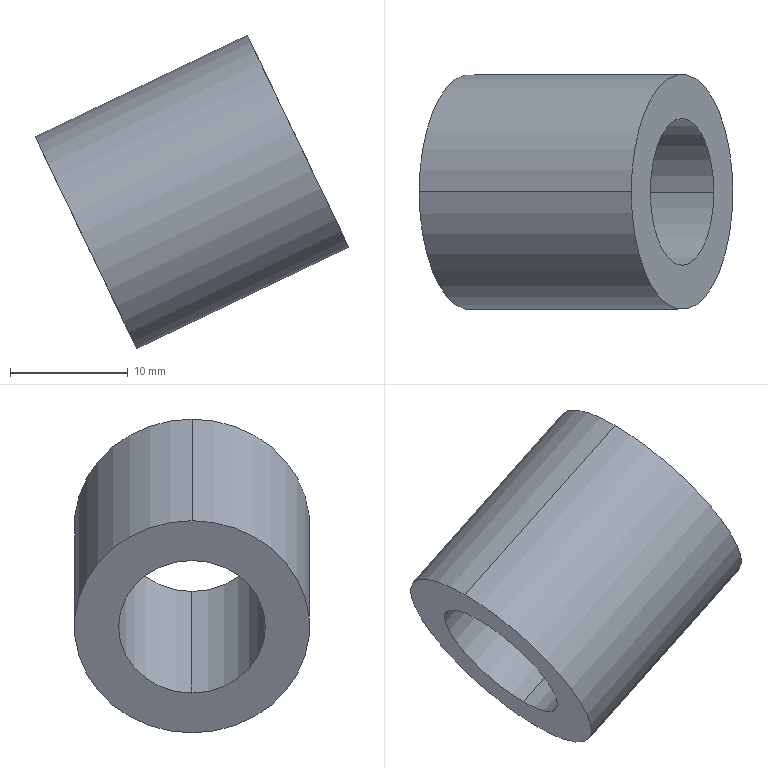Component | SolidWorks | Washer1-1-2 | 1 solid | 6 faces | box 26.68 x 20 x 26.68 mm | volume 3829 mm3 | cylinder 4 | plane 2 | commonest cylinder face diameters 12.5 x2 20 x2
build123d program:
from build123d import *

# Parameters (mm, degrees)
SKETCH1_R           = 10
SKETCH1_R_2         = 6.25
BOSS_EXTRUDE1_DEPTH = 20


with BuildPart() as part:
    # Sketch1 → Boss-Extrude1 (new body)
    with BuildSketch(Plane.XY):
        Circle(SKETCH1_R)
        Circle(SKETCH1_R_2, mode=Mode.SUBTRACT)
    extrude(amount=BOSS_EXTRUDE1_DEPTH)


solid = part.part

# Placed as in the assembly
solid = solid.moved(Location((-95.293, 250, 667.757), (0, 64.419, 168.667)))
STEP:
#1=COLOUR_RGB('',0.7922,0.8196,0.9333);
#2=FILL_AREA_STYLE_COLOUR('',#1);
#3=FILL_AREA_STYLE('',(#2));
#4=SURFACE_STYLE_FILL_AREA(#3);
#5=SURFACE_SIDE_STYLE('',(#4));
#6=SURFACE_STYLE_USAGE(.BOTH.,#5);
#7=PRESENTATION_STYLE_ASSIGNMENT((#6));
#8=CARTESIAN_POINT('',(-3.148,9.843,26.852));
#9=VERTEX_POINT('',#8);
#10=CARTESIAN_POINT('',(-2.935,9.843,26.408));
#11=VERTEX_POINT('',#10);
#12=CARTESIAN_POINT('',(-3.041,9.843,26.63));
#13=DIRECTION('',(0.902,-0.,0.4318));
#14=DIRECTION('',(0.4318,0.,-0.902));
#15=AXIS2_PLACEMENT_3D('',#12,#13,#14);
#16=CIRCLE('',#15,0.2461);
#17=EDGE_CURVE('',#9,#11,#16,.T.);
#18=ORIENTED_EDGE('',*,*,#17,.T.);
#19=CARTESIAN_POINT('',(-3.645,9.843,26.068));
#20=VERTEX_POINT('',#19);
#21=CARTESIAN_POINT('',(-2.935,9.843,26.408));
#22=DIRECTION('',(-0.902,0.,-0.4318));
#23=VECTOR('',#22,39.37);
#24=LINE('',#21,#23);
#25=EDGE_CURVE('',#11,#20,#24,.T.);
#26=ORIENTED_EDGE('',*,*,#25,.T.);
#27=CARTESIAN_POINT('',(-3.858,9.843,26.512));
#28=VERTEX_POINT('',#27);
#29=CARTESIAN_POINT('',(-3.752,9.843,26.29));
#30=DIRECTION('',(0.902,-0.,0.4318));
#31=DIRECTION('',(0.4318,0.,-0.902));
#32=AXIS2_PLACEMENT_3D('',#29,#30,#31);
#33=CIRCLE('',#32,0.2461);
#34=EDGE_CURVE('',#28,#20,#33,.T.);
#35=ORIENTED_EDGE('',*,*,#34,.F.);
#36=CARTESIAN_POINT('',(-3.148,9.843,26.852));
#37=DIRECTION('',(-0.902,0.,-0.4318));
#38=VECTOR('',#37,39.37);
#39=LINE('',#36,#38);
#40=EDGE_CURVE('',#9,#28,#39,.T.);
#41=ORIENTED_EDGE('',*,*,#40,.F.);
#42=EDGE_LOOP('',(#18,#26,#35,#41));
#43=FACE_OUTER_BOUND('',#42,.T.);
#44=CARTESIAN_POINT('',(-3.041,9.843,26.63));
#45=DIRECTION('',(-0.902,0.,-0.4318));
#46=DIRECTION('',(-0.4318,-0.,0.902));
#47=AXIS2_PLACEMENT_3D('',#44,#45,#46);
#48=CYLINDRICAL_SURFACE('',#47,0.2461);
#49=ADVANCED_FACE('',(#43),#48,.F.);
#50=CARTESIAN_POINT('',(-2.871,9.843,26.275));
#51=VERTEX_POINT('',#50);
#52=CARTESIAN_POINT('',(-3.211,9.843,26.985));
#53=VERTEX_POINT('',#52);
#54=CARTESIAN_POINT('',(-3.041,9.843,26.63));
#55=DIRECTION('',(0.902,-0.,0.4318));
#56=DIRECTION('',(0.4318,0.,-0.902));
#57=AXIS2_PLACEMENT_3D('',#54,#55,#56);
#58=CIRCLE('',#57,0.3937);
#59=EDGE_CURVE('',#51,#53,#58,.T.);
#60=ORIENTED_EDGE('',*,*,#59,.F.);
#61=CARTESIAN_POINT('',(-3.582,9.843,25.935));
#62=VERTEX_POINT('',#61);
#63=CARTESIAN_POINT('',(-2.871,9.843,26.275));
#64=DIRECTION('',(-0.902,0.,-0.4318));
#65=VECTOR('',#64,39.37);
#66=LINE('',#63,#65);
#67=EDGE_CURVE('',#51,#62,#66,.T.);
#68=ORIENTED_EDGE('',*,*,#67,.T.);
#69=CARTESIAN_POINT('',(-3.922,9.843,26.645));
#70=VERTEX_POINT('',#69);
#71=CARTESIAN_POINT('',(-3.752,9.843,26.29));
#72=DIRECTION('',(0.902,-0.,0.4318));
#73=DIRECTION('',(0.4318,0.,-0.902));
#74=AXIS2_PLACEMENT_3D('',#71,#72,#73);
#75=CIRCLE('',#74,0.3937);
#76=EDGE_CURVE('',#62,#70,#75,.T.);
#77=ORIENTED_EDGE('',*,*,#76,.T.);
#78=CARTESIAN_POINT('',(-3.211,9.843,26.985));
#79=DIRECTION('',(-0.902,0.,-0.4318));
#80=VECTOR('',#79,39.37);
#81=LINE('',#78,#80);
#82=EDGE_CURVE('',#53,#70,#81,.T.);
#83=ORIENTED_EDGE('',*,*,#82,.F.);
#84=EDGE_LOOP('',(#60,#68,#77,#83));
#85=FACE_OUTER_BOUND('',#84,.T.);
#86=CARTESIAN_POINT('',(-3.041,9.843,26.63));
#87=DIRECTION('',(-0.902,0.,-0.4318));
#88=DIRECTION('',(-0.4318,-0.,0.902));
#89=AXIS2_PLACEMENT_3D('',#86,#87,#88);
#90=CYLINDRICAL_SURFACE('',#89,0.3937);
#91=ADVANCED_FACE('',(#85),#90,.T.);
#92=CARTESIAN_POINT('',(-3.041,9.843,26.63));
#93=DIRECTION('',(0.902,-0.,0.4318));
#94=DIRECTION('',(0.4318,0.,-0.902));
#95=AXIS2_PLACEMENT_3D('',#92,#93,#94);
#96=CIRCLE('',#95,0.3937);
#97=EDGE_CURVE('',#53,#51,#96,.T.);
#98=ORIENTED_EDGE('',*,*,#97,.T.);
#99=ORIENTED_EDGE('',*,*,#59,.T.);
#100=EDGE_LOOP('',(#98,#99));
#101=FACE_OUTER_BOUND('',#100,.T.);
#102=ORIENTED_EDGE('',*,*,#17,.F.);
#103=CARTESIAN_POINT('',(-3.041,9.843,26.63));
#104=DIRECTION('',(0.902,-0.,0.4318));
#105=DIRECTION('',(0.4318,0.,-0.902));
#106=AXIS2_PLACEMENT_3D('',#103,#104,#105);
#107=CIRCLE('',#106,0.2461);
#108=EDGE_CURVE('',#11,#9,#107,.T.);
#109=ORIENTED_EDGE('',*,*,#108,.F.);
#110=EDGE_LOOP('',(#102,#109));
#111=FACE_BOUND('',#110,.T.);
#112=CARTESIAN_POINT('',(-3.041,9.843,26.63));
#113=DIRECTION('',(0.902,-0.,0.4318));
#114=DIRECTION('',(0.4318,0.,-0.902));
#115=AXIS2_PLACEMENT_3D('',#112,#113,#114);
#116=PLANE('',#115);
#117=ADVANCED_FACE('',(#101,#111),#116,.T.);
#118=CARTESIAN_POINT('',(-3.752,9.843,26.29));
#119=DIRECTION('',(0.902,-0.,0.4318));
#120=DIRECTION('',(0.4318,0.,-0.902));
#121=AXIS2_PLACEMENT_3D('',#118,#119,#120);
#122=CIRCLE('',#121,0.3937);
#123=EDGE_CURVE('',#70,#62,#122,.T.);
#124=ORIENTED_EDGE('',*,*,#123,.F.);
#125=ORIENTED_EDGE('',*,*,#76,.F.);
#126=EDGE_LOOP('',(#124,#125));
#127=FACE_OUTER_BOUND('',#126,.T.);
#128=ORIENTED_EDGE('',*,*,#34,.T.);
#129=CARTESIAN_POINT('',(-3.752,9.843,26.29));
#130=DIRECTION('',(0.902,-0.,0.4318));
#131=DIRECTION('',(0.4318,0.,-0.902));
#132=AXIS2_PLACEMENT_3D('',#129,#130,#131);
#133=CIRCLE('',#132,0.2461);
#134=EDGE_CURVE('',#20,#28,#133,.T.);
#135=ORIENTED_EDGE('',*,*,#134,.T.);
#136=EDGE_LOOP('',(#128,#135));
#137=FACE_BOUND('',#136,.T.);
#138=CARTESIAN_POINT('',(-3.752,9.843,26.29));
#139=DIRECTION('',(0.902,-0.,0.4318));
#140=DIRECTION('',(0.4318,0.,-0.902));
#141=AXIS2_PLACEMENT_3D('',#138,#139,#140);
#142=PLANE('',#141);
#143=ADVANCED_FACE('',(#127,#137),#142,.F.);
#144=ORIENTED_EDGE('',*,*,#67,.F.);
#145=ORIENTED_EDGE('',*,*,#97,.F.);
#146=ORIENTED_EDGE('',*,*,#82,.T.);
#147=ORIENTED_EDGE('',*,*,#123,.T.);
#148=EDGE_LOOP('',(#144,#145,#146,#147));
#149=FACE_OUTER_BOUND('',#148,.T.);
#150=CARTESIAN_POINT('',(-3.041,9.843,26.63));
#151=DIRECTION('',(-0.902,0.,-0.4318));
#152=DIRECTION('',(-0.4318,-0.,0.902));
#153=AXIS2_PLACEMENT_3D('',#150,#151,#152);
#154=CYLINDRICAL_SURFACE('',#153,0.3937);
#155=ADVANCED_FACE('',(#149),#154,.T.);
#156=ORIENTED_EDGE('',*,*,#25,.F.);
#157=ORIENTED_EDGE('',*,*,#108,.T.);
#158=ORIENTED_EDGE('',*,*,#40,.T.);
#159=ORIENTED_EDGE('',*,*,#134,.F.);
#160=EDGE_LOOP('',(#156,#157,#158,#159));
#161=FACE_OUTER_BOUND('',#160,.T.);
#162=CARTESIAN_POINT('',(-3.041,9.843,26.63));
#163=DIRECTION('',(-0.902,0.,-0.4318));
#164=DIRECTION('',(-0.4318,-0.,0.902));
#165=AXIS2_PLACEMENT_3D('',#162,#163,#164);
#166=CYLINDRICAL_SURFACE('',#165,0.2461);
#167=ADVANCED_FACE('',(#161),#166,.F.);
#168=CLOSED_SHELL('',(#49,#91,#117,#143,#155,#167));
#169=MANIFOLD_SOLID_BREP('',#168);
#170=STYLED_ITEM('',(#7),#169);
#171=PRESENTATION_LAYER_ASSIGNMENT('','',(#170));
#172=(LENGTH_UNIT()NAMED_UNIT(*)SI_UNIT($,.METRE.));
#173=LENGTH_MEASURE_WITH_UNIT(LENGTH_MEASURE(0.0254),#172);
#174=DIMENSIONAL_EXPONENTS(1.,0.,0.,0.,0.,0.,0.);
#175=(CONVERSION_BASED_UNIT('',#173)LENGTH_UNIT()NAMED_UNIT(#174));
#176=UNCERTAINTY_MEASURE_WITH_UNIT(LENGTH_MEASURE(0.00001),#175,'','');
#177=(NAMED_UNIT(*)PLANE_ANGLE_UNIT()SI_UNIT($,.RADIAN.));
#178=(NAMED_UNIT(*)SI_UNIT($,.STERADIAN.)SOLID_ANGLE_UNIT());
#179=(GEOMETRIC_REPRESENTATION_CONTEXT(3)GLOBAL_UNCERTAINTY_ASSIGNED_CONTEXT((#176))GLOBAL_UNIT_ASSIGNED_CONTEXT((#175,#177,#178))REPRESENTATION_CONTEXT('',''));
#180=MECHANICAL_DESIGN_GEOMETRIC_PRESENTATION_REPRESENTATION('',(#170),#179);
#181=CARTESIAN_POINT('',(0.,0.,0.));
#182=DIRECTION('',(0.,0.,1.));
#183=DIRECTION('',(1.,0.,0.));
#184=AXIS2_PLACEMENT_3D('',#181,#182,#183);
#185=(LENGTH_UNIT()NAMED_UNIT(*)SI_UNIT($,.METRE.));
#186=LENGTH_MEASURE_WITH_UNIT(LENGTH_MEASURE(0.0254),#185);
#187=DIMENSIONAL_EXPONENTS(1.,0.,0.,0.,0.,0.,0.);
#188=(CONVERSION_BASED_UNIT('',#186)LENGTH_UNIT()NAMED_UNIT(#187));
#189=UNCERTAINTY_MEASURE_WITH_UNIT(LENGTH_MEASURE(0.00001),#188,'','');
#190=(NAMED_UNIT(*)PLANE_ANGLE_UNIT()SI_UNIT($,.RADIAN.));
#191=(NAMED_UNIT(*)SI_UNIT($,.STERADIAN.)SOLID_ANGLE_UNIT());
#192=(GEOMETRIC_REPRESENTATION_CONTEXT(3)GLOBAL_UNCERTAINTY_ASSIGNED_CONTEXT((#189))GLOBAL_UNIT_ASSIGNED_CONTEXT((#188,#190,#191))REPRESENTATION_CONTEXT('',''));
#193=ADVANCED_BREP_SHAPE_REPRESENTATION('',(#169,#184),#192);